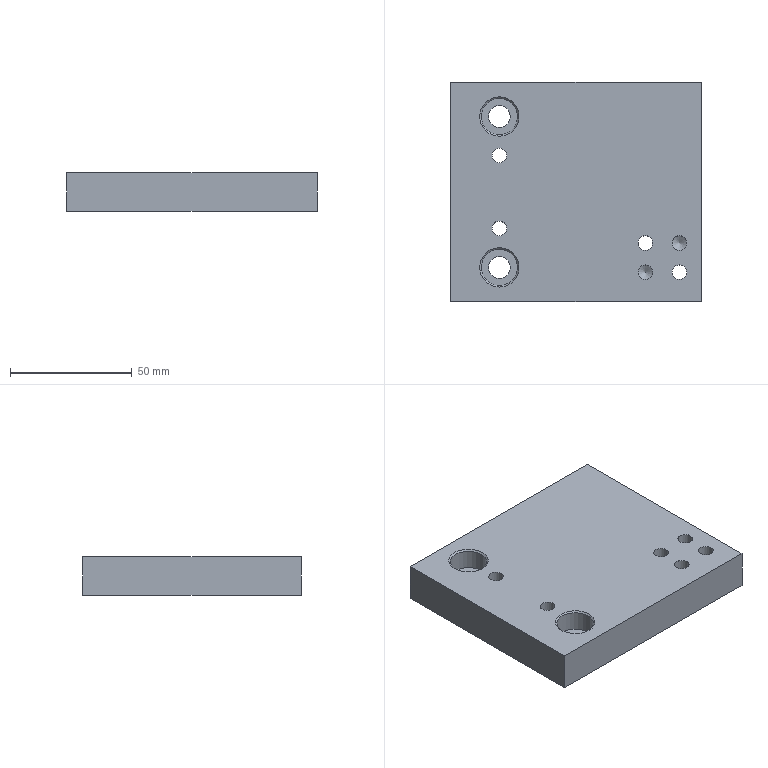Component | NX | SHIM_BLOCK | 1 solid | 26 faces | volume 141782 mm3 | cylinder 10 | plane 8 | cone 8 | commonest cylinder face diameters 6 x4 9 x2 15 x2 5.9 x2